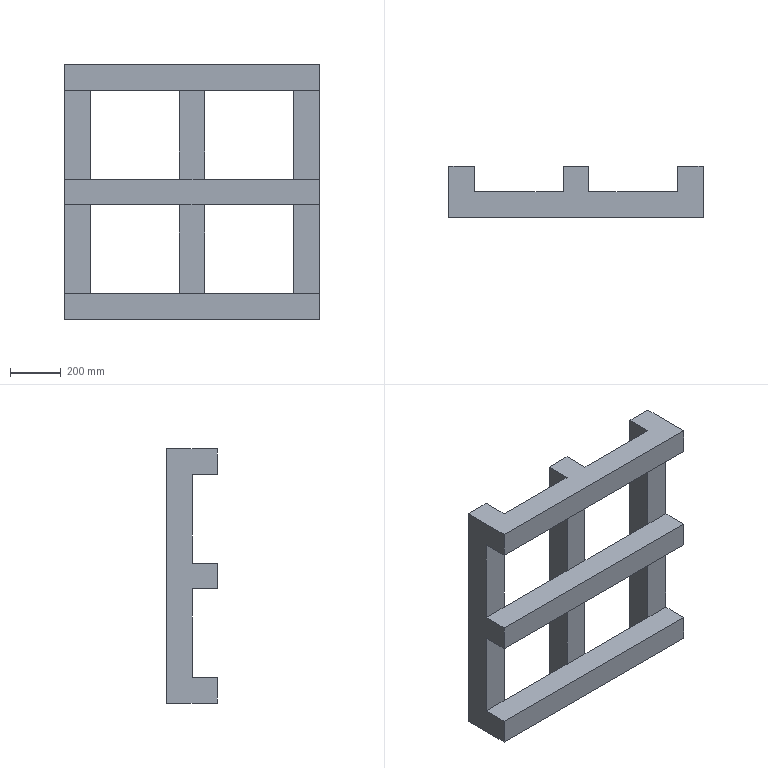Component | SolidWorks | WoodenFrameBase-1 | 1 solid | 30 faces | box 1000 x 200 x 1000 mm | volume 60000000 mm3 | plane 30
build123d program:
from build123d import *

# Parameters (mm, degrees)
SKETCH1_W             = 100
SKETCH1_H             = 1000
BOSS_EXTRUDE1_DEPTH   = 100
BOSS_EXTRUDE1_2_DEPTH = 100
BOSS_EXTRUDE1_3_DEPTH = 100
SKETCH3_W             = 1000
SKETCH3_H             = 100
BOSS_EXTRUDE3_DEPTH   = 100


with BuildPart() as part:
    # Sketch1 → Boss-Extrude1 (new body)
    with BuildSketch(Plane(origin=(0, 0, 0), x_dir=(1, 0, 0), z_dir=(0, 1, 0))):
        Rectangle(SKETCH1_W, SKETCH1_H)
    extrude(amount=BOSS_EXTRUDE1_DEPTH)



with BuildPart() as body_2:
    # Sketch1 → Boss-Extrude1 2 (new body)
    with BuildSketch(Plane(origin=(0, 0, 0), x_dir=(1, 0, 0), z_dir=(0, 1, 0))):
        with Locations((450, 0)):
            Rectangle(SKETCH1_W, SKETCH1_H)
    extrude(amount=BOSS_EXTRUDE1_2_DEPTH)


with BuildPart() as body_3:
    # Sketch1 → Boss-Extrude1 3 (new body)
    with BuildSketch(Plane(origin=(0, 0, 0), x_dir=(1, 0, 0), z_dir=(0, 1, 0))):
        with Locations((-450, 0)):
            Rectangle(SKETCH1_W, SKETCH1_H)
    extrude(amount=BOSS_EXTRUDE1_3_DEPTH)


with BuildPart() as part_1:
    add(part.part)

    add(body_2.part)  # Boss-Extrude3 merges body 2

    add(body_3.part)  # Boss-Extrude3 merges body 3
    # Sketch3 → Boss-Extrude3 (add)
    with BuildSketch(Plane.XZ):
        with Locations((0, 450)):
            Rectangle(SKETCH3_W, SKETCH3_H)
        Rectangle(SKETCH3_W, SKETCH3_H)
        with Locations((0, -450)):
            Rectangle(SKETCH3_W, SKETCH3_H)
    extrude(amount=BOSS_EXTRUDE3_DEPTH)


solid = part_1.part
STEP:
#1=COLOUR_RGB('',0.7922,0.8196,0.9333);
#2=FILL_AREA_STYLE_COLOUR('',#1);
#3=FILL_AREA_STYLE('',(#2));
#4=SURFACE_STYLE_FILL_AREA(#3);
#5=SURFACE_SIDE_STYLE('',(#4));
#6=SURFACE_STYLE_USAGE(.BOTH.,#5);
#7=PRESENTATION_STYLE_ASSIGNMENT((#6));
#8=CARTESIAN_POINT('',(1.969,0.,-15.748));
#9=VERTEX_POINT('',#8);
#10=CARTESIAN_POINT('',(-1.969,0.,-15.748));
#11=VERTEX_POINT('',#10);
#12=CARTESIAN_POINT('',(19.685,0.,-15.748));
#13=DIRECTION('',(-1.,0.,-0.));
#14=VECTOR('',#13,39.37);
#15=LINE('',#12,#14);
#16=EDGE_CURVE('',#9,#11,#15,.T.);
#17=ORIENTED_EDGE('',*,*,#16,.F.);
#18=CARTESIAN_POINT('',(1.969,0.,-1.969));
#19=VERTEX_POINT('',#18);
#20=CARTESIAN_POINT('',(1.969,0.,-0.));
#21=DIRECTION('',(0.,0.,1.));
#22=VECTOR('',#21,39.37);
#23=LINE('',#20,#22);
#24=EDGE_CURVE('',#9,#19,#23,.T.);
#25=ORIENTED_EDGE('',*,*,#24,.T.);
#26=CARTESIAN_POINT('',(-1.969,0.,-1.969));
#27=VERTEX_POINT('',#26);
#28=CARTESIAN_POINT('',(-19.685,0.,-1.969));
#29=DIRECTION('',(1.,0.,0.));
#30=VECTOR('',#29,39.37);
#31=LINE('',#28,#30);
#32=EDGE_CURVE('',#27,#19,#31,.T.);
#33=ORIENTED_EDGE('',*,*,#32,.F.);
#34=CARTESIAN_POINT('',(-1.969,0.,0.));
#35=DIRECTION('',(0.,0.,1.));
#36=VECTOR('',#35,39.37);
#37=LINE('',#34,#36);
#38=EDGE_CURVE('',#11,#27,#37,.T.);
#39=ORIENTED_EDGE('',*,*,#38,.F.);
#40=EDGE_LOOP('',(#17,#25,#33,#39));
#41=FACE_OUTER_BOUND('',#40,.T.);
#42=CARTESIAN_POINT('',(0.,0.,0.));
#43=DIRECTION('',(0.,1.,0.));
#44=DIRECTION('',(0.,0.,1.));
#45=AXIS2_PLACEMENT_3D('',#42,#43,#44);
#46=PLANE('',#45);
#47=ADVANCED_FACE('',(#41),#46,.F.);
#48=CARTESIAN_POINT('',(19.685,0.,-15.748));
#49=VERTEX_POINT('',#48);
#50=CARTESIAN_POINT('',(15.748,0.,-15.748));
#51=VERTEX_POINT('',#50);
#52=CARTESIAN_POINT('',(19.685,0.,-15.748));
#53=DIRECTION('',(-1.,0.,-0.));
#54=VECTOR('',#53,39.37);
#55=LINE('',#52,#54);
#56=EDGE_CURVE('',#49,#51,#55,.T.);
#57=ORIENTED_EDGE('',*,*,#56,.F.);
#58=CARTESIAN_POINT('',(19.685,0.,-1.969));
#59=VERTEX_POINT('',#58);
#60=CARTESIAN_POINT('',(19.685,0.,0.));
#61=DIRECTION('',(0.,0.,1.));
#62=VECTOR('',#61,39.37);
#63=LINE('',#60,#62);
#64=EDGE_CURVE('',#49,#59,#63,.T.);
#65=ORIENTED_EDGE('',*,*,#64,.T.);
#66=CARTESIAN_POINT('',(15.748,0.,-1.969));
#67=VERTEX_POINT('',#66);
#68=CARTESIAN_POINT('',(-19.685,0.,-1.969));
#69=DIRECTION('',(1.,0.,0.));
#70=VECTOR('',#69,39.37);
#71=LINE('',#68,#70);
#72=EDGE_CURVE('',#67,#59,#71,.T.);
#73=ORIENTED_EDGE('',*,*,#72,.F.);
#74=CARTESIAN_POINT('',(15.748,0.,0.));
#75=DIRECTION('',(0.,0.,1.));
#76=VECTOR('',#75,39.37);
#77=LINE('',#74,#76);
#78=EDGE_CURVE('',#51,#67,#77,.T.);
#79=ORIENTED_EDGE('',*,*,#78,.F.);
#80=EDGE_LOOP('',(#57,#65,#73,#79));
#81=FACE_OUTER_BOUND('',#80,.T.);
#82=CARTESIAN_POINT('',(0.,0.,0.));
#83=DIRECTION('',(0.,1.,0.));
#84=DIRECTION('',(0.,0.,1.));
#85=AXIS2_PLACEMENT_3D('',#82,#83,#84);
#86=PLANE('',#85);
#87=ADVANCED_FACE('',(#81),#86,.F.);
#88=CARTESIAN_POINT('',(-15.748,0.,-15.748));
#89=VERTEX_POINT('',#88);
#90=CARTESIAN_POINT('',(-19.685,0.,-15.748));
#91=VERTEX_POINT('',#90);
#92=CARTESIAN_POINT('',(19.685,0.,-15.748));
#93=DIRECTION('',(-1.,0.,-0.));
#94=VECTOR('',#93,39.37);
#95=LINE('',#92,#94);
#96=EDGE_CURVE('',#89,#91,#95,.T.);
#97=ORIENTED_EDGE('',*,*,#96,.F.);
#98=CARTESIAN_POINT('',(-15.748,0.,-1.969));
#99=VERTEX_POINT('',#98);
#100=CARTESIAN_POINT('',(-15.748,0.,-19.685));
#101=DIRECTION('',(0.,0.,1.));
#102=VECTOR('',#101,39.37);
#103=LINE('',#100,#102);
#104=EDGE_CURVE('',#89,#99,#103,.T.);
#105=ORIENTED_EDGE('',*,*,#104,.T.);
#106=CARTESIAN_POINT('',(-19.685,0.,-1.969));
#107=VERTEX_POINT('',#106);
#108=CARTESIAN_POINT('',(-19.685,0.,-1.969));
#109=DIRECTION('',(1.,0.,0.));
#110=VECTOR('',#109,39.37);
#111=LINE('',#108,#110);
#112=EDGE_CURVE('',#107,#99,#111,.T.);
#113=ORIENTED_EDGE('',*,*,#112,.F.);
#114=CARTESIAN_POINT('',(-19.685,0.,-19.685));
#115=DIRECTION('',(0.,0.,1.));
#116=VECTOR('',#115,39.37);
#117=LINE('',#114,#116);
#118=EDGE_CURVE('',#91,#107,#117,.T.);
#119=ORIENTED_EDGE('',*,*,#118,.F.);
#120=EDGE_LOOP('',(#97,#105,#113,#119));
#121=FACE_OUTER_BOUND('',#120,.T.);
#122=CARTESIAN_POINT('',(0.,0.,0.));
#123=DIRECTION('',(0.,1.,0.));
#124=DIRECTION('',(0.,0.,1.));
#125=AXIS2_PLACEMENT_3D('',#122,#123,#124);
#126=PLANE('',#125);
#127=ADVANCED_FACE('',(#121),#126,.F.);
#128=CARTESIAN_POINT('',(1.969,0.,1.969));
#129=VERTEX_POINT('',#128);
#130=CARTESIAN_POINT('',(-1.969,0.,1.969));
#131=VERTEX_POINT('',#130);
#132=CARTESIAN_POINT('',(19.685,0.,1.969));
#133=DIRECTION('',(-1.,0.,-0.));
#134=VECTOR('',#133,39.37);
#135=LINE('',#132,#134);
#136=EDGE_CURVE('',#129,#131,#135,.T.);
#137=ORIENTED_EDGE('',*,*,#136,.F.);
#138=CARTESIAN_POINT('',(1.969,0.,15.748));
#139=VERTEX_POINT('',#138);
#140=CARTESIAN_POINT('',(1.969,0.,-0.));
#141=DIRECTION('',(0.,0.,1.));
#142=VECTOR('',#141,39.37);
#143=LINE('',#140,#142);
#144=EDGE_CURVE('',#129,#139,#143,.T.);
#145=ORIENTED_EDGE('',*,*,#144,.T.);
#146=CARTESIAN_POINT('',(-1.969,0.,15.748));
#147=VERTEX_POINT('',#146);
#148=CARTESIAN_POINT('',(-19.685,0.,15.748));
#149=DIRECTION('',(1.,0.,0.));
#150=VECTOR('',#149,39.37);
#151=LINE('',#148,#150);
#152=EDGE_CURVE('',#147,#139,#151,.T.);
#153=ORIENTED_EDGE('',*,*,#152,.F.);
#154=CARTESIAN_POINT('',(-1.969,0.,0.));
#155=DIRECTION('',(0.,0.,1.));
#156=VECTOR('',#155,39.37);
#157=LINE('',#154,#156);
#158=EDGE_CURVE('',#131,#147,#157,.T.);
#159=ORIENTED_EDGE('',*,*,#158,.F.);
#160=EDGE_LOOP('',(#137,#145,#153,#159));
#161=FACE_OUTER_BOUND('',#160,.T.);
#162=CARTESIAN_POINT('',(0.,0.,0.));
#163=DIRECTION('',(0.,1.,0.));
#164=DIRECTION('',(0.,0.,1.));
#165=AXIS2_PLACEMENT_3D('',#162,#163,#164);
#166=PLANE('',#165);
#167=ADVANCED_FACE('',(#161),#166,.F.);
#168=CARTESIAN_POINT('',(19.685,0.,1.969));
#169=VERTEX_POINT('',#168);
#170=CARTESIAN_POINT('',(15.748,0.,1.969));
#171=VERTEX_POINT('',#170);
#172=CARTESIAN_POINT('',(19.685,0.,1.969));
#173=DIRECTION('',(-1.,0.,-0.));
#174=VECTOR('',#173,39.37);
#175=LINE('',#172,#174);
#176=EDGE_CURVE('',#169,#171,#175,.T.);
#177=ORIENTED_EDGE('',*,*,#176,.F.);
#178=CARTESIAN_POINT('',(19.685,0.,15.748));
#179=VERTEX_POINT('',#178);
#180=CARTESIAN_POINT('',(19.685,0.,0.));
#181=DIRECTION('',(0.,0.,1.));
#182=VECTOR('',#181,39.37);
#183=LINE('',#180,#182);
#184=EDGE_CURVE('',#169,#179,#183,.T.);
#185=ORIENTED_EDGE('',*,*,#184,.T.);
#186=CARTESIAN_POINT('',(15.748,0.,15.748));
#187=VERTEX_POINT('',#186);
#188=CARTESIAN_POINT('',(-19.685,0.,15.748));
#189=DIRECTION('',(-1.,0.,-0.));
#190=VECTOR('',#189,39.37);
#191=LINE('',#188,#190);
#192=EDGE_CURVE('',#179,#187,#191,.T.);
#193=ORIENTED_EDGE('',*,*,#192,.T.);
#194=CARTESIAN_POINT('',(15.748,0.,0.));
#195=DIRECTION('',(0.,0.,1.));
#196=VECTOR('',#195,39.37);
#197=LINE('',#194,#196);
#198=EDGE_CURVE('',#171,#187,#197,.T.);
#199=ORIENTED_EDGE('',*,*,#198,.F.);
#200=EDGE_LOOP('',(#177,#185,#193,#199));
#201=FACE_OUTER_BOUND('',#200,.T.);
#202=CARTESIAN_POINT('',(0.,0.,0.));
#203=DIRECTION('',(0.,1.,0.));
#204=DIRECTION('',(0.,0.,1.));
#205=AXIS2_PLACEMENT_3D('',#202,#203,#204);
#206=PLANE('',#205);
#207=ADVANCED_FACE('',(#201),#206,.F.);
#208=CARTESIAN_POINT('',(-15.748,0.,1.969));
#209=VERTEX_POINT('',#208);
#210=CARTESIAN_POINT('',(-19.685,0.,1.969));
#211=VERTEX_POINT('',#210);
#212=CARTESIAN_POINT('',(19.685,0.,1.969));
#213=DIRECTION('',(-1.,0.,-0.));
#214=VECTOR('',#213,39.37);
#215=LINE('',#212,#214);
#216=EDGE_CURVE('',#209,#211,#215,.T.);
#217=ORIENTED_EDGE('',*,*,#216,.F.);
#218=CARTESIAN_POINT('',(-15.748,0.,15.748));
#219=VERTEX_POINT('',#218);
#220=CARTESIAN_POINT('',(-15.748,0.,-19.685));
#221=DIRECTION('',(0.,0.,1.));
#222=VECTOR('',#221,39.37);
#223=LINE('',#220,#222);
#224=EDGE_CURVE('',#209,#219,#223,.T.);
#225=ORIENTED_EDGE('',*,*,#224,.T.);
#226=CARTESIAN_POINT('',(-19.685,0.,15.748));
#227=VERTEX_POINT('',#226);
#228=CARTESIAN_POINT('',(-19.685,0.,15.748));
#229=DIRECTION('',(1.,0.,0.));
#230=VECTOR('',#229,39.37);
#231=LINE('',#228,#230);
#232=EDGE_CURVE('',#227,#219,#231,.T.);
#233=ORIENTED_EDGE('',*,*,#232,.F.);
#234=CARTESIAN_POINT('',(-19.685,0.,-19.685));
#235=DIRECTION('',(0.,0.,1.));
#236=VECTOR('',#235,39.37);
#237=LINE('',#234,#236);
#238=EDGE_CURVE('',#211,#227,#237,.T.);
#239=ORIENTED_EDGE('',*,*,#238,.F.);
#240=EDGE_LOOP('',(#217,#225,#233,#239));
#241=FACE_OUTER_BOUND('',#240,.T.);
#242=CARTESIAN_POINT('',(0.,0.,0.));
#243=DIRECTION('',(0.,1.,0.));
#244=DIRECTION('',(0.,0.,1.));
#245=AXIS2_PLACEMENT_3D('',#242,#243,#244);
#246=PLANE('',#245);
#247=ADVANCED_FACE('',(#241),#246,.F.);
#248=CARTESIAN_POINT('',(15.748,0.,19.685));
#249=VERTEX_POINT('',#248);
#250=CARTESIAN_POINT('',(15.748,0.,0.));
#251=DIRECTION('',(0.,0.,1.));
#252=VECTOR('',#251,39.37);
#253=LINE('',#250,#252);
#254=EDGE_CURVE('',#187,#249,#253,.T.);
#255=ORIENTED_EDGE('',*,*,#254,.F.);
#256=CARTESIAN_POINT('',(-19.685,0.,15.748));
#257=DIRECTION('',(1.,0.,0.));
#258=VECTOR('',#257,39.37);
#259=LINE('',#256,#258);
#260=EDGE_CURVE('',#139,#187,#259,.T.);
#261=ORIENTED_EDGE('',*,*,#260,.F.);
#262=CARTESIAN_POINT('',(1.969,0.,19.685));
#263=VERTEX_POINT('',#262);
#264=CARTESIAN_POINT('',(1.969,0.,-0.));
#265=DIRECTION('',(0.,0.,1.));
#266=VECTOR('',#265,39.37);
#267=LINE('',#264,#266);
#268=EDGE_CURVE('',#139,#263,#267,.T.);
#269=ORIENTED_EDGE('',*,*,#268,.T.);
#270=CARTESIAN_POINT('',(19.685,0.,19.685));
#271=DIRECTION('',(-1.,0.,-0.));
#272=VECTOR('',#271,39.37);
#273=LINE('',#270,#272);
#274=EDGE_CURVE('',#249,#263,#273,.T.);
#275=ORIENTED_EDGE('',*,*,#274,.F.);
#276=EDGE_LOOP('',(#255,#261,#269,#275));
#277=FACE_OUTER_BOUND('',#276,.T.);
#278=CARTESIAN_POINT('',(0.,0.,0.));
#279=DIRECTION('',(0.,-1.,0.));
#280=DIRECTION('',(0.,0.,-1.));
#281=AXIS2_PLACEMENT_3D('',#278,#279,#280);
#282=PLANE('',#281);
#283=ADVANCED_FACE('',(#277),#282,.F.);
#284=CARTESIAN_POINT('',(1.969,3.937,-19.685));
#285=VERTEX_POINT('',#284);
#286=CARTESIAN_POINT('',(1.969,0.,-19.685));
#287=VERTEX_POINT('',#286);
#288=CARTESIAN_POINT('',(1.969,3.937,-19.685));
#289=DIRECTION('',(0.,-1.,0.));
#290=VECTOR('',#289,39.37);
#291=LINE('',#288,#290);
#292=EDGE_CURVE('',#285,#287,#291,.T.);
#293=ORIENTED_EDGE('',*,*,#292,.T.);
#294=CARTESIAN_POINT('',(15.748,0.,-19.685));
#295=VERTEX_POINT('',#294);
#296=CARTESIAN_POINT('',(-19.685,0.,-19.685));
#297=DIRECTION('',(1.,0.,0.));
#298=VECTOR('',#297,39.37);
#299=LINE('',#296,#298);
#300=EDGE_CURVE('',#287,#295,#299,.T.);
#301=ORIENTED_EDGE('',*,*,#300,.T.);
#302=CARTESIAN_POINT('',(15.748,3.937,-19.685));
#303=VERTEX_POINT('',#302);
#304=CARTESIAN_POINT('',(15.748,3.937,-19.685));
#305=DIRECTION('',(0.,-1.,0.));
#306=VECTOR('',#305,39.37);
#307=LINE('',#304,#306);
#308=EDGE_CURVE('',#303,#295,#307,.T.);
#309=ORIENTED_EDGE('',*,*,#308,.F.);
#310=CARTESIAN_POINT('',(19.685,3.937,-19.685));
#311=VERTEX_POINT('',#310);
#312=CARTESIAN_POINT('',(0.,3.937,-19.685));
#313=DIRECTION('',(-1.,0.,0.));
#314=VECTOR('',#313,39.37);
#315=LINE('',#312,#314);
#316=EDGE_CURVE('',#311,#303,#315,.T.);
#317=ORIENTED_EDGE('',*,*,#316,.F.);
#318=CARTESIAN_POINT('',(19.685,-3.937,-19.685));
#319=VERTEX_POINT('',#318);
#320=CARTESIAN_POINT('',(19.685,3.937,-19.685));
#321=DIRECTION('',(0.,-1.,0.));
#322=VECTOR('',#321,39.37);
#323=LINE('',#320,#322);
#324=EDGE_CURVE('',#311,#319,#323,.T.);
#325=ORIENTED_EDGE('',*,*,#324,.T.);
#326=CARTESIAN_POINT('',(-19.685,-3.937,-19.685));
#327=VERTEX_POINT('',#326);
#328=CARTESIAN_POINT('',(-19.685,-3.937,-19.685));
#329=DIRECTION('',(1.,0.,0.));
#330=VECTOR('',#329,39.37);
#331=LINE('',#328,#330);
#332=EDGE_CURVE('',#327,#319,#331,.T.);
#333=ORIENTED_EDGE('',*,*,#332,.F.);
#334=CARTESIAN_POINT('',(-19.685,3.937,-19.685));
#335=VERTEX_POINT('',#334);
#336=CARTESIAN_POINT('',(-19.685,3.937,-19.685));
#337=DIRECTION('',(0.,-1.,0.));
#338=VECTOR('',#337,39.37);
#339=LINE('',#336,#338);
#340=EDGE_CURVE('',#335,#327,#339,.T.);
#341=ORIENTED_EDGE('',*,*,#340,.F.);
#342=CARTESIAN_POINT('',(-15.748,3.937,-19.685));
#343=VERTEX_POINT('',#342);
#344=CARTESIAN_POINT('',(-15.748,3.937,-19.685));
#345=DIRECTION('',(-1.,0.,0.));
#346=VECTOR('',#345,39.37);
#347=LINE('',#344,#346);
#348=EDGE_CURVE('',#343,#335,#347,.T.);
#349=ORIENTED_EDGE('',*,*,#348,.F.);
#350=CARTESIAN_POINT('',(-15.748,0.,-19.685));
#351=VERTEX_POINT('',#350);
#352=CARTESIAN_POINT('',(-15.748,3.937,-19.685));
#353=DIRECTION('',(0.,-1.,0.));
#354=VECTOR('',#353,39.37);
#355=LINE('',#352,#354);
#356=EDGE_CURVE('',#343,#351,#355,.T.);
#357=ORIENTED_EDGE('',*,*,#356,.T.);
#358=CARTESIAN_POINT('',(-1.969,0.,-19.685));
#359=VERTEX_POINT('',#358);
#360=CARTESIAN_POINT('',(-19.685,0.,-19.685));
#361=DIRECTION('',(1.,0.,0.));
#362=VECTOR('',#361,39.37);
#363=LINE('',#360,#362);
#364=EDGE_CURVE('',#351,#359,#363,.T.);
#365=ORIENTED_EDGE('',*,*,#364,.T.);
#366=CARTESIAN_POINT('',(-1.969,3.937,-19.685));
#367=VERTEX_POINT('',#366);
#368=CARTESIAN_POINT('',(-1.969,3.937,-19.685));
#369=DIRECTION('',(0.,-1.,0.));
#370=VECTOR('',#369,39.37);
#371=LINE('',#368,#370);
#372=EDGE_CURVE('',#367,#359,#371,.T.);
#373=ORIENTED_EDGE('',*,*,#372,.F.);
#374=CARTESIAN_POINT('',(-0.,3.937,-19.685));
#375=DIRECTION('',(-1.,0.,0.));
#376=VECTOR('',#375,39.37);
#377=LINE('',#374,#376);
#378=EDGE_CURVE('',#285,#367,#377,.T.);
#379=ORIENTED_EDGE('',*,*,#378,.F.);
#380=EDGE_LOOP('',(#293,#301,#309,#317,#325,#333,#341,#349,#357,#365,#373,#379));
#381=FACE_OUTER_BOUND('',#380,.T.);
#382=CARTESIAN_POINT('',(-0.,3.937,-19.685));
#383=DIRECTION('',(0.,0.,1.));
#384=DIRECTION('',(1.,0.,-0.));
#385=AXIS2_PLACEMENT_3D('',#382,#383,#384);
#386=PLANE('',#385);
#387=ADVANCED_FACE('',(#381),#386,.F.);
#388=CARTESIAN_POINT('',(-1.969,0.,0.));
#389=DIRECTION('',(0.,0.,1.));
#390=VECTOR('',#389,39.37);
#391=LINE('',#388,#390);
#392=EDGE_CURVE('',#359,#11,#391,.T.);
#393=ORIENTED_EDGE('',*,*,#392,.T.);
#394=ORIENTED_EDGE('',*,*,#38,.T.);
#395=CARTESIAN_POINT('',(-1.969,0.,0.));
#396=DIRECTION('',(-0.,0.,-1.));
#397=VECTOR('',#396,39.37);
#398=LINE('',#395,#397);
#399=EDGE_CURVE('',#131,#27,#398,.T.);
#400=ORIENTED_EDGE('',*,*,#399,.F.);
#401=ORIENTED_EDGE('',*,*,#158,.T.);
#402=CARTESIAN_POINT('',(-1.969,0.,19.685));
#403=VERTEX_POINT('',#402);
#404=CARTESIAN_POINT('',(-1.969,0.,0.));
#405=DIRECTION('',(0.,0.,1.));
#406=VECTOR('',#405,39.37);
#407=LINE('',#404,#406);
#408=EDGE_CURVE('',#147,#403,#407,.T.);
#409=ORIENTED_EDGE('',*,*,#408,.T.);
#410=CARTESIAN_POINT('',(-1.969,3.937,19.685));
#411=VERTEX_POINT('',#410);
#412=CARTESIAN_POINT('',(-1.969,3.937,19.685));
#413=DIRECTION('',(0.,-1.,0.));
#414=VECTOR('',#413,39.37);
#415=LINE('',#412,#414);
#416=EDGE_CURVE('',#411,#403,#415,.T.);
#417=ORIENTED_EDGE('',*,*,#416,.F.);
#418=CARTESIAN_POINT('',(-1.969,3.937,0.));
#419=DIRECTION('',(0.,0.,1.));
#420=VECTOR('',#419,39.37);
#421=LINE('',#418,#420);
#422=EDGE_CURVE('',#367,#411,#421,.T.);
#423=ORIENTED_EDGE('',*,*,#422,.F.);
#424=ORIENTED_EDGE('',*,*,#372,.T.);
#425=EDGE_LOOP('',(#393,#394,#400,#401,#409,#417,#423,#424));
#426=FACE_OUTER_BOUND('',#425,.T.);
#427=CARTESIAN_POINT('',(-1.969,3.937,0.));
#428=DIRECTION('',(1.,0.,-0.));
#429=DIRECTION('',(-0.,0.,-1.));
#430=AXIS2_PLACEMENT_3D('',#427,#428,#429);
#431=PLANE('',#430);
#432=ADVANCED_FACE('',(#426),#431,.F.);
#433=ORIENTED_EDGE('',*,*,#416,.T.);
#434=CARTESIAN_POINT('',(-15.748,0.,19.685));
#435=VERTEX_POINT('',#434);
#436=CARTESIAN_POINT('',(19.685,0.,19.685));
#437=DIRECTION('',(-1.,0.,-0.));
#438=VECTOR('',#437,39.37);
#439=LINE('',#436,#438);
#440=EDGE_CURVE('',#403,#435,#439,.T.);
#441=ORIENTED_EDGE('',*,*,#440,.T.);
#442=CARTESIAN_POINT('',(-15.748,3.937,19.685));
#443=VERTEX_POINT('',#442);
#444=CARTESIAN_POINT('',(-15.748,3.937,19.685));
#445=DIRECTION('',(0.,-1.,0.));
#446=VECTOR('',#445,39.37);
#447=LINE('',#444,#446);
#448=EDGE_CURVE('',#443,#435,#447,.T.);
#449=ORIENTED_EDGE('',*,*,#448,.F.);
#450=CARTESIAN_POINT('',(-19.685,3.937,19.685));
#451=VERTEX_POINT('',#450);
#452=CARTESIAN_POINT('',(-15.748,3.937,19.685));
#453=DIRECTION('',(-1.,0.,0.));
#454=VECTOR('',#453,39.37);
#455=LINE('',#452,#454);
#456=EDGE_CURVE('',#443,#451,#455,.T.);
#457=ORIENTED_EDGE('',*,*,#456,.T.);
#458=CARTESIAN_POINT('',(-19.685,-3.937,19.685));
#459=VERTEX_POINT('',#458);
#460=CARTESIAN_POINT('',(-19.685,-3.937,19.685));
#461=DIRECTION('',(0.,1.,0.));
#462=VECTOR('',#461,39.37);
#463=LINE('',#460,#462);
#464=EDGE_CURVE('',#459,#451,#463,.T.);
#465=ORIENTED_EDGE('',*,*,#464,.F.);
#466=CARTESIAN_POINT('',(19.685,-3.937,19.685));
#467=VERTEX_POINT('',#466);
#468=CARTESIAN_POINT('',(19.685,-3.937,19.685));
#469=DIRECTION('',(-1.,0.,-0.));
#470=VECTOR('',#469,39.37);
#471=LINE('',#468,#470);
#472=EDGE_CURVE('',#467,#459,#471,.T.);
#473=ORIENTED_EDGE('',*,*,#472,.F.);
#474=CARTESIAN_POINT('',(19.685,3.937,19.685));
#475=VERTEX_POINT('',#474);
#476=CARTESIAN_POINT('',(19.685,-3.937,19.685));
#477=DIRECTION('',(0.,1.,0.));
#478=VECTOR('',#477,39.37);
#479=LINE('',#476,#478);
#480=EDGE_CURVE('',#467,#475,#479,.T.);
#481=ORIENTED_EDGE('',*,*,#480,.T.);
#482=CARTESIAN_POINT('',(15.748,3.937,19.685));
#483=VERTEX_POINT('',#482);
#484=CARTESIAN_POINT('',(0.,3.937,19.685));
#485=DIRECTION('',(-1.,0.,0.));
#486=VECTOR('',#485,39.37);
#487=LINE('',#484,#486);
#488=EDGE_CURVE('',#475,#483,#487,.T.);
#489=ORIENTED_EDGE('',*,*,#488,.T.);
#490=CARTESIAN_POINT('',(15.748,3.937,19.685));
#491=DIRECTION('',(0.,-1.,0.));
#492=VECTOR('',#491,39.37);
#493=LINE('',#490,#492);
#494=EDGE_CURVE('',#483,#249,#493,.T.);
#495=ORIENTED_EDGE('',*,*,#494,.T.);
#496=ORIENTED_EDGE('',*,*,#274,.T.);
#497=CARTESIAN_POINT('',(1.969,3.937,19.685));
#498=VERTEX_POINT('',#497);
#499=CARTESIAN_POINT('',(1.969,3.937,19.685));
#500=DIRECTION('',(0.,-1.,0.));
#501=VECTOR('',#500,39.37);
#502=LINE('',#499,#501);
#503=EDGE_CURVE('',#498,#263,#502,.T.);
#504=ORIENTED_EDGE('',*,*,#503,.F.);
#505=CARTESIAN_POINT('',(0.,3.937,19.685));
#506=DIRECTION('',(-1.,0.,0.));
#507=VECTOR('',#506,39.37);
#508=LINE('',#505,#507);
#509=EDGE_CURVE('',#498,#411,#508,.T.);
#510=ORIENTED_EDGE('',*,*,#509,.T.);
#511=EDGE_LOOP('',(#433,#441,#449,#457,#465,#473,#481,#489,#495,#496,#504,#510));
#512=FACE_OUTER_BOUND('',#511,.T.);
#513=CARTESIAN_POINT('',(0.,3.937,19.685));
#514=DIRECTION('',(0.,0.,1.));
#515=DIRECTION('',(1.,0.,0.));
#516=AXIS2_PLACEMENT_3D('',#513,#514,#515);
#517=PLANE('',#516);
#518=ADVANCED_FACE('',(#512),#517,.T.);
#519=CARTESIAN_POINT('',(1.969,0.,-0.));
#520=DIRECTION('',(0.,0.,1.));
#521=VECTOR('',#520,39.37);
#522=LINE('',#519,#521);
#523=EDGE_CURVE('',#287,#9,#522,.T.);
#524=ORIENTED_EDGE('',*,*,#523,.F.);
#525=ORIENTED_EDGE('',*,*,#292,.F.);
#526=CARTESIAN_POINT('',(1.969,3.937,-0.));
#527=DIRECTION('',(0.,0.,1.));
#528=VECTOR('',#527,39.37);
#529=LINE('',#526,#528);
#530=EDGE_CURVE('',#285,#498,#529,.T.);
#531=ORIENTED_EDGE('',*,*,#530,.T.);
#532=ORIENTED_EDGE('',*,*,#503,.T.);
#533=ORIENTED_EDGE('',*,*,#268,.F.);
#534=ORIENTED_EDGE('',*,*,#144,.F.);
#535=CARTESIAN_POINT('',(1.969,0.,-0.));
#536=DIRECTION('',(-0.,0.,-1.));
#537=VECTOR('',#536,39.37);
#538=LINE('',#535,#537);
#539=EDGE_CURVE('',#129,#19,#538,.T.);
#540=ORIENTED_EDGE('',*,*,#539,.T.);
#541=ORIENTED_EDGE('',*,*,#24,.F.);
#542=EDGE_LOOP('',(#524,#525,#531,#532,#533,#534,#540,#541));
#543=FACE_OUTER_BOUND('',#542,.T.);
#544=CARTESIAN_POINT('',(1.969,3.937,-0.));
#545=DIRECTION('',(1.,0.,-0.));
#546=DIRECTION('',(-0.,0.,-1.));
#547=AXIS2_PLACEMENT_3D('',#544,#545,#546);
#548=PLANE('',#547);
#549=ADVANCED_FACE('',(#543),#548,.T.);
#550=ORIENTED_EDGE('',*,*,#378,.T.);
#551=ORIENTED_EDGE('',*,*,#422,.T.);
#552=ORIENTED_EDGE('',*,*,#509,.F.);
#553=ORIENTED_EDGE('',*,*,#530,.F.);
#554=EDGE_LOOP('',(#550,#551,#552,#553));
#555=FACE_OUTER_BOUND('',#554,.T.);
#556=CARTESIAN_POINT('',(0.,3.937,0.));
#557=DIRECTION('',(0.,1.,0.));
#558=DIRECTION('',(0.,0.,1.));
#559=AXIS2_PLACEMENT_3D('',#556,#557,#558);
#560=PLANE('',#559);
#561=ADVANCED_FACE('',(#555),#560,.T.);
#562=ORIENTED_EDGE('',*,*,#232,.T.);
#563=CARTESIAN_POINT('',(-19.685,0.,15.748));
#564=DIRECTION('',(1.,0.,0.));
#565=VECTOR('',#564,39.37);
#566=LINE('',#563,#565);
#567=EDGE_CURVE('',#219,#147,#566,.T.);
#568=ORIENTED_EDGE('',*,*,#567,.T.);
#569=ORIENTED_EDGE('',*,*,#152,.T.);
#570=ORIENTED_EDGE('',*,*,#260,.T.);
#571=ORIENTED_EDGE('',*,*,#192,.F.);
#572=CARTESIAN_POINT('',(19.685,-3.937,15.748));
#573=VERTEX_POINT('',#572);
#574=CARTESIAN_POINT('',(19.685,-3.937,15.748));
#575=DIRECTION('',(0.,1.,0.));
#576=VECTOR('',#575,39.37);
#577=LINE('',#574,#576);
#578=EDGE_CURVE('',#573,#179,#577,.T.);
#579=ORIENTED_EDGE('',*,*,#578,.F.);
#580=CARTESIAN_POINT('',(-19.685,-3.937,15.748));
#581=VERTEX_POINT('',#580);
#582=CARTESIAN_POINT('',(-19.685,-3.937,15.748));
#583=DIRECTION('',(1.,0.,0.));
#584=VECTOR('',#583,39.37);
#585=LINE('',#582,#584);
#586=EDGE_CURVE('',#581,#573,#585,.T.);
#587=ORIENTED_EDGE('',*,*,#586,.F.);
#588=CARTESIAN_POINT('',(-19.685,-3.937,15.748));
#589=DIRECTION('',(0.,1.,0.));
#590=VECTOR('',#589,39.37);
#591=LINE('',#588,#590);
#592=EDGE_CURVE('',#581,#227,#591,.T.);
#593=ORIENTED_EDGE('',*,*,#592,.T.);
#594=EDGE_LOOP('',(#562,#568,#569,#570,#571,#579,#587,#593));
#595=FACE_OUTER_BOUND('',#594,.T.);
#596=CARTESIAN_POINT('',(-19.685,-3.937,15.748));
#597=DIRECTION('',(-0.,0.,1.));
#598=DIRECTION('',(1.,0.,0.));
#599=AXIS2_PLACEMENT_3D('',#596,#597,#598);
#600=PLANE('',#599);
#601=ADVANCED_FACE('',(#595),#600,.F.);
#602=ORIENTED_EDGE('',*,*,#578,.T.);
#603=ORIENTED_EDGE('',*,*,#184,.F.);
#604=CARTESIAN_POINT('',(19.685,-3.937,1.969));
#605=VERTEX_POINT('',#604);
#606=CARTESIAN_POINT('',(19.685,-3.937,1.969));
#607=DIRECTION('',(0.,1.,0.));
#608=VECTOR('',#607,39.37);
#609=LINE('',#606,#608);
#610=EDGE_CURVE('',#605,#169,#609,.T.);
#611=ORIENTED_EDGE('',*,*,#610,.F.);
#612=CARTESIAN_POINT('',(19.685,-3.937,-1.969));
#613=VERTEX_POINT('',#612);
#614=CARTESIAN_POINT('',(19.685,-3.937,-1.969));
#615=DIRECTION('',(-0.,0.,1.));
#616=VECTOR('',#615,39.37);
#617=LINE('',#614,#616);
#618=EDGE_CURVE('',#613,#605,#617,.T.);
#619=ORIENTED_EDGE('',*,*,#618,.F.);
#620=CARTESIAN_POINT('',(19.685,-3.937,-1.969));
#621=DIRECTION('',(0.,1.,0.));
#622=VECTOR('',#621,39.37);
#623=LINE('',#620,#622);
#624=EDGE_CURVE('',#613,#59,#623,.T.);
#625=ORIENTED_EDGE('',*,*,#624,.T.);
#626=ORIENTED_EDGE('',*,*,#64,.F.);
#627=CARTESIAN_POINT('',(19.685,-3.937,-15.748));
#628=VERTEX_POINT('',#627);
#629=CARTESIAN_POINT('',(19.685,-3.937,-15.748));
#630=DIRECTION('',(0.,1.,0.));
#631=VECTOR('',#630,39.37);
#632=LINE('',#629,#631);
#633=EDGE_CURVE('',#628,#49,#632,.T.);
#634=ORIENTED_EDGE('',*,*,#633,.F.);
#635=CARTESIAN_POINT('',(19.685,-3.937,-19.685));
#636=DIRECTION('',(-0.,0.,1.));
#637=VECTOR('',#636,39.37);
#638=LINE('',#635,#637);
#639=EDGE_CURVE('',#319,#628,#638,.T.);
#640=ORIENTED_EDGE('',*,*,#639,.F.);
#641=ORIENTED_EDGE('',*,*,#324,.F.);
#642=CARTESIAN_POINT('',(19.685,3.937,0.));
#643=DIRECTION('',(0.,0.,1.));
#644=VECTOR('',#643,39.37);
#645=LINE('',#642,#644);
#646=EDGE_CURVE('',#311,#475,#645,.T.);
#647=ORIENTED_EDGE('',*,*,#646,.T.);
#648=ORIENTED_EDGE('',*,*,#480,.F.);
#649=CARTESIAN_POINT('',(19.685,-3.937,15.748));
#650=DIRECTION('',(-0.,0.,1.));
#651=VECTOR('',#650,39.37);
#652=LINE('',#649,#651);
#653=EDGE_CURVE('',#573,#467,#652,.T.);
#654=ORIENTED_EDGE('',*,*,#653,.F.);
#655=EDGE_LOOP('',(#602,#603,#611,#619,#625,#626,#634,#640,#641,#647,#648,#654));
#656=FACE_OUTER_BOUND('',#655,.T.);
#657=CARTESIAN_POINT('',(19.685,-3.937,15.748));
#658=DIRECTION('',(-1.,0.,-0.));
#659=DIRECTION('',(-0.,0.,1.));
#660=AXIS2_PLACEMENT_3D('',#657,#658,#659);
#661=PLANE('',#660);
#662=ADVANCED_FACE('',(#656),#661,.F.);
#663=ORIENTED_EDGE('',*,*,#464,.T.);
#664=CARTESIAN_POINT('',(-19.685,3.937,-19.685));
#665=DIRECTION('',(0.,0.,1.));
#666=VECTOR('',#665,39.37);
#667=LINE('',#664,#666);
#668=EDGE_CURVE('',#335,#451,#667,.T.);
#669=ORIENTED_EDGE('',*,*,#668,.F.);
#670=ORIENTED_EDGE('',*,*,#340,.T.);
#671=CARTESIAN_POINT('',(-19.685,-3.937,-15.748));
#672=VERTEX_POINT('',#671);
#673=CARTESIAN_POINT('',(-19.685,-3.937,-15.748));
#674=DIRECTION('',(0.,0.,-1.));
#675=VECTOR('',#674,39.37);
#676=LINE('',#673,#675);
#677=EDGE_CURVE('',#672,#327,#676,.T.);
#678=ORIENTED_EDGE('',*,*,#677,.F.);
#679=CARTESIAN_POINT('',(-19.685,-3.937,-15.748));
#680=DIRECTION('',(0.,1.,0.));
#681=VECTOR('',#680,39.37);
#682=LINE('',#679,#681);
#683=EDGE_CURVE('',#672,#91,#682,.T.);
#684=ORIENTED_EDGE('',*,*,#683,.T.);
#685=ORIENTED_EDGE('',*,*,#118,.T.);
#686=CARTESIAN_POINT('',(-19.685,-3.937,-1.969));
#687=VERTEX_POINT('',#686);
#688=CARTESIAN_POINT('',(-19.685,-3.937,-1.969));
#689=DIRECTION('',(0.,1.,0.));
#690=VECTOR('',#689,39.37);
#691=LINE('',#688,#690);
#692=EDGE_CURVE('',#687,#107,#691,.T.);
#693=ORIENTED_EDGE('',*,*,#692,.F.);
#694=CARTESIAN_POINT('',(-19.685,-3.937,1.969));
#695=VERTEX_POINT('',#694);
#696=CARTESIAN_POINT('',(-19.685,-3.937,1.969));
#697=DIRECTION('',(0.,0.,-1.));
#698=VECTOR('',#697,39.37);
#699=LINE('',#696,#698);
#700=EDGE_CURVE('',#695,#687,#699,.T.);
#701=ORIENTED_EDGE('',*,*,#700,.F.);
#702=CARTESIAN_POINT('',(-19.685,-3.937,1.969));
#703=DIRECTION('',(0.,1.,0.));
#704=VECTOR('',#703,39.37);
#705=LINE('',#702,#704);
#706=EDGE_CURVE('',#695,#211,#705,.T.);
#707=ORIENTED_EDGE('',*,*,#706,.T.);
#708=ORIENTED_EDGE('',*,*,#238,.T.);
#709=ORIENTED_EDGE('',*,*,#592,.F.);
#710=CARTESIAN_POINT('',(-19.685,-3.937,19.685));
#711=DIRECTION('',(0.,0.,-1.));
#712=VECTOR('',#711,39.37);
#713=LINE('',#710,#712);
#714=EDGE_CURVE('',#459,#581,#713,.T.);
#715=ORIENTED_EDGE('',*,*,#714,.F.);
#716=EDGE_LOOP('',(#663,#669,#670,#678,#684,#685,#693,#701,#707,#708,#709,#715));
#717=FACE_OUTER_BOUND('',#716,.T.);
#718=CARTESIAN_POINT('',(-19.685,-3.937,19.685));
#719=DIRECTION('',(1.,0.,0.));
#720=DIRECTION('',(0.,0.,-1.));
#721=AXIS2_PLACEMENT_3D('',#718,#719,#720);
#722=PLANE('',#721);
#723=ADVANCED_FACE('',(#717),#722,.F.);
#724=ORIENTED_EDGE('',*,*,#586,.T.);
#725=ORIENTED_EDGE('',*,*,#653,.T.);
#726=ORIENTED_EDGE('',*,*,#472,.T.);
#727=ORIENTED_EDGE('',*,*,#714,.T.);
#728=EDGE_LOOP('',(#724,#725,#726,#727));
#729=FACE_OUTER_BOUND('',#728,.T.);
#730=CARTESIAN_POINT('',(0.,-3.937,0.));
#731=DIRECTION('',(0.,-1.,0.));
#732=DIRECTION('',(0.,0.,-1.));
#733=AXIS2_PLACEMENT_3D('',#730,#731,#732);
#734=PLANE('',#733);
#735=ADVANCED_FACE('',(#729),#734,.T.);
#736=ORIENTED_EDGE('',*,*,#567,.F.);
#737=CARTESIAN_POINT('',(-15.748,0.,0.));
#738=DIRECTION('',(0.,0.,1.));
#739=VECTOR('',#738,39.37);
#740=LINE('',#737,#739);
#741=EDGE_CURVE('',#219,#435,#740,.T.);
#742=ORIENTED_EDGE('',*,*,#741,.T.);
#743=ORIENTED_EDGE('',*,*,#440,.F.);
#744=ORIENTED_EDGE('',*,*,#408,.F.);
#745=EDGE_LOOP('',(#736,#742,#743,#744));
#746=FACE_OUTER_BOUND('',#745,.T.);
#747=CARTESIAN_POINT('',(0.,0.,0.));
#748=DIRECTION('',(0.,-1.,0.));
#749=DIRECTION('',(0.,0.,-1.));
#750=AXIS2_PLACEMENT_3D('',#747,#748,#749);
#751=PLANE('',#750);
#752=ADVANCED_FACE('',(#746),#751,.F.);
#753=CARTESIAN_POINT('',(15.748,0.,0.));
#754=DIRECTION('',(0.,0.,1.));
#755=VECTOR('',#754,39.37);
#756=LINE('',#753,#755);
#757=EDGE_CURVE('',#295,#51,#756,.T.);
#758=ORIENTED_EDGE('',*,*,#757,.T.);
#759=ORIENTED_EDGE('',*,*,#78,.T.);
#760=CARTESIAN_POINT('',(15.748,0.,0.));
#761=DIRECTION('',(0.,0.,-1.));
#762=VECTOR('',#761,39.37);
#763=LINE('',#760,#762);
#764=EDGE_CURVE('',#171,#67,#763,.T.);
#765=ORIENTED_EDGE('',*,*,#764,.F.);
#766=ORIENTED_EDGE('',*,*,#198,.T.);
#767=ORIENTED_EDGE('',*,*,#254,.T.);
#768=ORIENTED_EDGE('',*,*,#494,.F.);
#769=CARTESIAN_POINT('',(15.748,3.937,0.));
#770=DIRECTION('',(0.,0.,1.));
#771=VECTOR('',#770,39.37);
#772=LINE('',#769,#771);
#773=EDGE_CURVE('',#303,#483,#772,.T.);
#774=ORIENTED_EDGE('',*,*,#773,.F.);
#775=ORIENTED_EDGE('',*,*,#308,.T.);
#776=EDGE_LOOP('',(#758,#759,#765,#766,#767,#768,#774,#775));
#777=FACE_OUTER_BOUND('',#776,.T.);
#778=CARTESIAN_POINT('',(15.748,3.937,0.));
#779=DIRECTION('',(1.,0.,0.));
#780=DIRECTION('',(0.,0.,-1.));
#781=AXIS2_PLACEMENT_3D('',#778,#779,#780);
#782=PLANE('',#781);
#783=ADVANCED_FACE('',(#777),#782,.F.);
#784=ORIENTED_EDGE('',*,*,#316,.T.);
#785=ORIENTED_EDGE('',*,*,#773,.T.);
#786=ORIENTED_EDGE('',*,*,#488,.F.);
#787=ORIENTED_EDGE('',*,*,#646,.F.);
#788=EDGE_LOOP('',(#784,#785,#786,#787));
#789=FACE_OUTER_BOUND('',#788,.T.);
#790=CARTESIAN_POINT('',(0.,3.937,0.));
#791=DIRECTION('',(0.,1.,0.));
#792=DIRECTION('',(0.,0.,1.));
#793=AXIS2_PLACEMENT_3D('',#790,#791,#792);
#794=PLANE('',#793);
#795=ADVANCED_FACE('',(#789),#794,.T.);
#796=CARTESIAN_POINT('',(-15.748,0.,-19.685));
#797=DIRECTION('',(0.,0.,1.));
#798=VECTOR('',#797,39.37);
#799=LINE('',#796,#798);
#800=EDGE_CURVE('',#351,#89,#799,.T.);
#801=ORIENTED_EDGE('',*,*,#800,.F.);
#802=ORIENTED_EDGE('',*,*,#356,.F.);
#803=CARTESIAN_POINT('',(-15.748,3.937,-19.685));
#804=DIRECTION('',(0.,0.,1.));
#805=VECTOR('',#804,39.37);
#806=LINE('',#803,#805);
#807=EDGE_CURVE('',#343,#443,#806,.T.);
#808=ORIENTED_EDGE('',*,*,#807,.T.);
#809=ORIENTED_EDGE('',*,*,#448,.T.);
#810=ORIENTED_EDGE('',*,*,#741,.F.);
#811=ORIENTED_EDGE('',*,*,#224,.F.);
#812=CARTESIAN_POINT('',(-15.748,0.,-19.685));
#813=DIRECTION('',(0.,0.,1.));
#814=VECTOR('',#813,39.37);
#815=LINE('',#812,#814);
#816=EDGE_CURVE('',#99,#209,#815,.T.);
#817=ORIENTED_EDGE('',*,*,#816,.F.);
#818=ORIENTED_EDGE('',*,*,#104,.F.);
#819=EDGE_LOOP('',(#801,#802,#808,#809,#810,#811,#817,#818));
#820=FACE_OUTER_BOUND('',#819,.T.);
#821=CARTESIAN_POINT('',(-15.748,3.937,-19.685));
#822=DIRECTION('',(1.,0.,-0.));
#823=DIRECTION('',(-0.,0.,-1.));
#824=AXIS2_PLACEMENT_3D('',#821,#822,#823);
#825=PLANE('',#824);
#826=ADVANCED_FACE('',(#820),#825,.T.);
#827=ORIENTED_EDGE('',*,*,#348,.T.);
#828=ORIENTED_EDGE('',*,*,#668,.T.);
#829=ORIENTED_EDGE('',*,*,#456,.F.);
#830=ORIENTED_EDGE('',*,*,#807,.F.);
#831=EDGE_LOOP('',(#827,#828,#829,#830));
#832=FACE_OUTER_BOUND('',#831,.T.);
#833=CARTESIAN_POINT('',(0.,3.937,0.));
#834=DIRECTION('',(0.,1.,0.));
#835=DIRECTION('',(0.,0.,1.));
#836=AXIS2_PLACEMENT_3D('',#833,#834,#835);
#837=PLANE('',#836);
#838=ADVANCED_FACE('',(#832),#837,.T.);
#839=CARTESIAN_POINT('',(19.685,0.,1.969));
#840=DIRECTION('',(-1.,0.,-0.));
#841=VECTOR('',#840,39.37);
#842=LINE('',#839,#841);
#843=EDGE_CURVE('',#131,#209,#842,.T.);
#844=ORIENTED_EDGE('',*,*,#843,.F.);
#845=ORIENTED_EDGE('',*,*,#399,.T.);
#846=CARTESIAN_POINT('',(-19.685,0.,-1.969));
#847=DIRECTION('',(1.,0.,0.));
#848=VECTOR('',#847,39.37);
#849=LINE('',#846,#848);
#850=EDGE_CURVE('',#99,#27,#849,.T.);
#851=ORIENTED_EDGE('',*,*,#850,.F.);
#852=ORIENTED_EDGE('',*,*,#816,.T.);
#853=EDGE_LOOP('',(#844,#845,#851,#852));
#854=FACE_OUTER_BOUND('',#853,.T.);
#855=CARTESIAN_POINT('',(0.,0.,0.));
#856=DIRECTION('',(0.,-1.,0.));
#857=DIRECTION('',(0.,0.,-1.));
#858=AXIS2_PLACEMENT_3D('',#855,#856,#857);
#859=PLANE('',#858);
#860=ADVANCED_FACE('',(#854),#859,.F.);
#861=ORIENTED_EDGE('',*,*,#539,.F.);
#862=CARTESIAN_POINT('',(19.685,0.,1.969));
#863=DIRECTION('',(-1.,0.,-0.));
#864=VECTOR('',#863,39.37);
#865=LINE('',#862,#864);
#866=EDGE_CURVE('',#171,#129,#865,.T.);
#867=ORIENTED_EDGE('',*,*,#866,.F.);
#868=ORIENTED_EDGE('',*,*,#764,.T.);
#869=CARTESIAN_POINT('',(-19.685,0.,-1.969));
#870=DIRECTION('',(1.,0.,0.));
#871=VECTOR('',#870,39.37);
#872=LINE('',#869,#871);
#873=EDGE_CURVE('',#19,#67,#872,.T.);
#874=ORIENTED_EDGE('',*,*,#873,.F.);
#875=EDGE_LOOP('',(#861,#867,#868,#874));
#876=FACE_OUTER_BOUND('',#875,.T.);
#877=CARTESIAN_POINT('',(0.,0.,0.));
#878=DIRECTION('',(0.,-1.,0.));
#879=DIRECTION('',(0.,0.,-1.));
#880=AXIS2_PLACEMENT_3D('',#877,#878,#879);
#881=PLANE('',#880);
#882=ADVANCED_FACE('',(#876),#881,.F.);
#883=ORIENTED_EDGE('',*,*,#112,.T.);
#884=ORIENTED_EDGE('',*,*,#850,.T.);
#885=ORIENTED_EDGE('',*,*,#32,.T.);
#886=ORIENTED_EDGE('',*,*,#873,.T.);
#887=ORIENTED_EDGE('',*,*,#72,.T.);
#888=ORIENTED_EDGE('',*,*,#624,.F.);
#889=CARTESIAN_POINT('',(-19.685,-3.937,-1.969));
#890=DIRECTION('',(1.,0.,0.));
#891=VECTOR('',#890,39.37);
#892=LINE('',#889,#891);
#893=EDGE_CURVE('',#687,#613,#892,.T.);
#894=ORIENTED_EDGE('',*,*,#893,.F.);
#895=ORIENTED_EDGE('',*,*,#692,.T.);
#896=EDGE_LOOP('',(#883,#884,#885,#886,#887,#888,#894,#895));
#897=FACE_OUTER_BOUND('',#896,.T.);
#898=CARTESIAN_POINT('',(-19.685,-3.937,-1.969));
#899=DIRECTION('',(-0.,0.,1.));
#900=DIRECTION('',(1.,0.,0.));
#901=AXIS2_PLACEMENT_3D('',#898,#899,#900);
#902=PLANE('',#901);
#903=ADVANCED_FACE('',(#897),#902,.F.);
#904=ORIENTED_EDGE('',*,*,#176,.T.);
#905=ORIENTED_EDGE('',*,*,#866,.T.);
#906=ORIENTED_EDGE('',*,*,#136,.T.);
#907=ORIENTED_EDGE('',*,*,#843,.T.);
#908=ORIENTED_EDGE('',*,*,#216,.T.);
#909=ORIENTED_EDGE('',*,*,#706,.F.);
#910=CARTESIAN_POINT('',(19.685,-3.937,1.969));
#911=DIRECTION('',(-1.,0.,-0.));
#912=VECTOR('',#911,39.37);
#913=LINE('',#910,#912);
#914=EDGE_CURVE('',#605,#695,#913,.T.);
#915=ORIENTED_EDGE('',*,*,#914,.F.);
#916=ORIENTED_EDGE('',*,*,#610,.T.);
#917=EDGE_LOOP('',(#904,#905,#906,#907,#908,#909,#915,#916));
#918=FACE_OUTER_BOUND('',#917,.T.);
#919=CARTESIAN_POINT('',(19.685,-3.937,1.969));
#920=DIRECTION('',(0.,0.,-1.));
#921=DIRECTION('',(-1.,0.,-0.));
#922=AXIS2_PLACEMENT_3D('',#919,#920,#921);
#923=PLANE('',#922);
#924=ADVANCED_FACE('',(#918),#923,.F.);
#925=ORIENTED_EDGE('',*,*,#893,.T.);
#926=ORIENTED_EDGE('',*,*,#618,.T.);
#927=ORIENTED_EDGE('',*,*,#914,.T.);
#928=ORIENTED_EDGE('',*,*,#700,.T.);
#929=EDGE_LOOP('',(#925,#926,#927,#928));
#930=FACE_OUTER_BOUND('',#929,.T.);
#931=CARTESIAN_POINT('',(0.,-3.937,0.));
#932=DIRECTION('',(0.,-1.,0.));
#933=DIRECTION('',(0.,0.,-1.));
#934=AXIS2_PLACEMENT_3D('',#931,#932,#933);
#935=PLANE('',#934);
#936=ADVANCED_FACE('',(#930),#935,.T.);
#937=CARTESIAN_POINT('',(19.685,0.,-15.748));
#938=DIRECTION('',(-1.,0.,-0.));
#939=VECTOR('',#938,39.37);
#940=LINE('',#937,#939);
#941=EDGE_CURVE('',#11,#89,#940,.T.);
#942=ORIENTED_EDGE('',*,*,#941,.F.);
#943=ORIENTED_EDGE('',*,*,#392,.F.);
#944=ORIENTED_EDGE('',*,*,#364,.F.);
#945=ORIENTED_EDGE('',*,*,#800,.T.);
#946=EDGE_LOOP('',(#942,#943,#944,#945));
#947=FACE_OUTER_BOUND('',#946,.T.);
#948=CARTESIAN_POINT('',(0.,0.,0.));
#949=DIRECTION('',(0.,-1.,0.));
#950=DIRECTION('',(0.,0.,-1.));
#951=AXIS2_PLACEMENT_3D('',#948,#949,#950);
#952=PLANE('',#951);
#953=ADVANCED_FACE('',(#947),#952,.F.);
#954=ORIENTED_EDGE('',*,*,#523,.T.);
#955=CARTESIAN_POINT('',(19.685,0.,-15.748));
#956=DIRECTION('',(-1.,0.,-0.));
#957=VECTOR('',#956,39.37);
#958=LINE('',#955,#957);
#959=EDGE_CURVE('',#51,#9,#958,.T.);
#960=ORIENTED_EDGE('',*,*,#959,.F.);
#961=ORIENTED_EDGE('',*,*,#757,.F.);
#962=ORIENTED_EDGE('',*,*,#300,.F.);
#963=EDGE_LOOP('',(#954,#960,#961,#962));
#964=FACE_OUTER_BOUND('',#963,.T.);
#965=CARTESIAN_POINT('',(0.,0.,0.));
#966=DIRECTION('',(0.,-1.,0.));
#967=DIRECTION('',(0.,0.,-1.));
#968=AXIS2_PLACEMENT_3D('',#965,#966,#967);
#969=PLANE('',#968);
#970=ADVANCED_FACE('',(#964),#969,.F.);
#971=ORIENTED_EDGE('',*,*,#56,.T.);
#972=ORIENTED_EDGE('',*,*,#959,.T.);
#973=ORIENTED_EDGE('',*,*,#16,.T.);
#974=ORIENTED_EDGE('',*,*,#941,.T.);
#975=ORIENTED_EDGE('',*,*,#96,.T.);
#976=ORIENTED_EDGE('',*,*,#683,.F.);
#977=CARTESIAN_POINT('',(19.685,-3.937,-15.748));
#978=DIRECTION('',(-1.,0.,-0.));
#979=VECTOR('',#978,39.37);
#980=LINE('',#977,#979);
#981=EDGE_CURVE('',#628,#672,#980,.T.);
#982=ORIENTED_EDGE('',*,*,#981,.F.);
#983=ORIENTED_EDGE('',*,*,#633,.T.);
#984=EDGE_LOOP('',(#971,#972,#973,#974,#975,#976,#982,#983));
#985=FACE_OUTER_BOUND('',#984,.T.);
#986=CARTESIAN_POINT('',(19.685,-3.937,-15.748));
#987=DIRECTION('',(0.,0.,-1.));
#988=DIRECTION('',(-1.,0.,-0.));
#989=AXIS2_PLACEMENT_3D('',#986,#987,#988);
#990=PLANE('',#989);
#991=ADVANCED_FACE('',(#985),#990,.F.);
#992=ORIENTED_EDGE('',*,*,#332,.T.);
#993=ORIENTED_EDGE('',*,*,#639,.T.);
#994=ORIENTED_EDGE('',*,*,#981,.T.);
#995=ORIENTED_EDGE('',*,*,#677,.T.);
#996=EDGE_LOOP('',(#992,#993,#994,#995));
#997=FACE_OUTER_BOUND('',#996,.T.);
#998=CARTESIAN_POINT('',(0.,-3.937,0.));
#999=DIRECTION('',(0.,-1.,0.));
#1000=DIRECTION('',(0.,0.,-1.));
#1001=AXIS2_PLACEMENT_3D('',#998,#999,#1000);
#1002=PLANE('',#1001);
#1003=ADVANCED_FACE('',(#997),#1002,.T.);
#1004=CLOSED_SHELL('',(#47,#87,#127,#167,#207,#247,#283,#387,#432,#518,#549,#561,#601,#662,#723,#735,#752,#783,#795,#826,#838,#860,#882,#903,#924,#936,#953,#970,#991,#1003));
#1005=MANIFOLD_SOLID_BREP('',#1004);
#1006=STYLED_ITEM('',(#7),#1005);
#1007=(LENGTH_UNIT()NAMED_UNIT(*)SI_UNIT($,.METRE.));
#1008=LENGTH_MEASURE_WITH_UNIT(LENGTH_MEASURE(0.0254),#1007);
#1009=DIMENSIONAL_EXPONENTS(1.,0.,0.,0.,0.,0.,0.);
#1010=(CONVERSION_BASED_UNIT('',#1008)LENGTH_UNIT()NAMED_UNIT(#1009));
#1011=UNCERTAINTY_MEASURE_WITH_UNIT(LENGTH_MEASURE(0.00001),#1010,'','');
#1012=(NAMED_UNIT(*)PLANE_ANGLE_UNIT()SI_UNIT($,.RADIAN.));
#1013=(NAMED_UNIT(*)SI_UNIT($,.STERADIAN.)SOLID_ANGLE_UNIT());
#1014=(GEOMETRIC_REPRESENTATION_CONTEXT(3)GLOBAL_UNCERTAINTY_ASSIGNED_CONTEXT((#1011))GLOBAL_UNIT_ASSIGNED_CONTEXT((#1010,#1012,#1013))REPRESENTATION_CONTEXT('',''));
#1015=MECHANICAL_DESIGN_GEOMETRIC_PRESENTATION_REPRESENTATION('',(#1006),#1014);
#1016=PRESENTATION_LAYER_ASSIGNMENT('','',(#1006));
#1017=CARTESIAN_POINT('',(0.,0.,0.));
#1018=DIRECTION('',(0.,0.,1.));
#1019=DIRECTION('',(1.,0.,0.));
#1020=AXIS2_PLACEMENT_3D('',#1017,#1018,#1019);
#1021=(LENGTH_UNIT()NAMED_UNIT(*)SI_UNIT($,.METRE.));
#1022=LENGTH_MEASURE_WITH_UNIT(LENGTH_MEASURE(0.0254),#1021);
#1023=DIMENSIONAL_EXPONENTS(1.,0.,0.,0.,0.,0.,0.);
#1024=(CONVERSION_BASED_UNIT('',#1022)LENGTH_UNIT()NAMED_UNIT(#1023));
#1025=UNCERTAINTY_MEASURE_WITH_UNIT(LENGTH_MEASURE(0.00001),#1024,'','');
#1026=(NAMED_UNIT(*)PLANE_ANGLE_UNIT()SI_UNIT($,.RADIAN.));
#1027=(NAMED_UNIT(*)SI_UNIT($,.STERADIAN.)SOLID_ANGLE_UNIT());
#1028=(GEOMETRIC_REPRESENTATION_CONTEXT(3)GLOBAL_UNCERTAINTY_ASSIGNED_CONTEXT((#1025))GLOBAL_UNIT_ASSIGNED_CONTEXT((#1024,#1026,#1027))REPRESENTATION_CONTEXT('',''));
#1029=ADVANCED_BREP_SHAPE_REPRESENTATION('',(#1005,#1020),#1028);